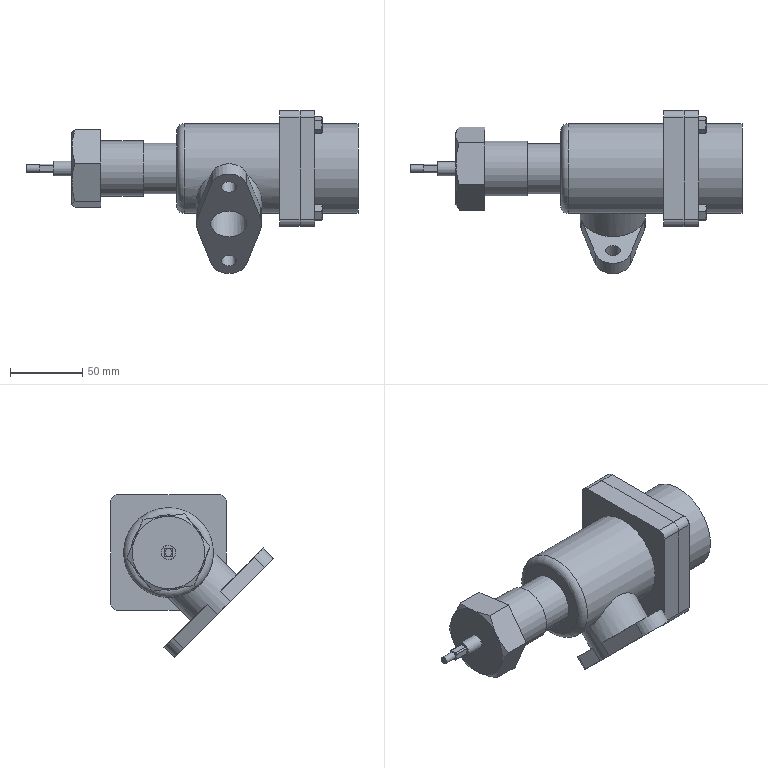Assembly | NX | mm | 19 component files | 19 solids | 279 faces | box 229 x 112.48 x 112.48 mm | volume 406841 mm3 | plane 116 | cylinder 79 | cone 79 | torus 3 | spline 1 | sphere 1 | commonest cylinder face diameters 6 x16 10 x13 16 x5 24 x4 2 x4 50 x3 40 x3 38 x3
Bill of materials:
GB-T6170_F-2000,M6x1 | 4 |  | Hexagonal prism with a central round through-bore; outer corners chamfered on both end faces; consistent with a hex nut form.
unnamed part 1 | 1 |  | Cylindrical plug or cap: a plain cylindrical body ending in a thin, tapered radial flange, followed by a short, smaller stepped disc that closes the end.
unnamed part 2 | 1 |  | Square flange with rounded corners and four corner holes. A larger hollow cylindrical boss sticks out from one face and two stepped, smaller cylindrical bosses stick out from the other face. A central round bore runs through.
unnamed part 3 | 1 |  | Flanged bushing: a thin annular flange with a smaller-diameter hollow cylindrical shank and a central through-bore.
unnamed part 4 | 1 |  | Flat circular ring with a rectangular cross-section, like a thin washer or spacer ring.
GB-T119.1-2000,6x24 | 4 |  | Parallel Pin, GB-T 119.1-2000,6x24
unnamed part 5 | 1 |  | Short thick-walled tubular sleeve with chamfered outer edges at both ends.
unnamed part 6 | 1 |  | Very thin flat annular ring, like a shim or thin washer.
unnamed part 7 | 1 |  | Housing body: a cylindrical main body with a square four-hole flange at one end, a stepped cylindrical spigot at the other end, and a side branch ending in an oval two-hole flange with a central bore, set at an angle.
unnamed part 8 | 1 |  | Slender stepped pin with a domed, hemispherical head at one end, a larger cylindrical collar near the head, and two reduced-diameter steps at the opposite tip.
unnamed part 9 | 1 |  | Hexagonal block with a large blind or stepped bore on one face and a smaller central through-hole visible from the opposite face. One end has chamfered corners.
unnamed part 10 | 1 |  | Thick flat annular ring or spacer with a rectangular cross-section.
unnamed part 11 | 1 |  | Hexagonal flange with a coaxial hollow cylindrical spigot. A short, narrower neck or undercut lies between the hex and the spigot, and a round through-bore runs through.
Mates:
1. touch align | valve_seat 1 face | valve_body 1 face
2. touch align | packing_gland 1 face | valve_body 1 face
3. touch align | gasket 1 face | valve_body 1 face
4. touch align | gasket 1 face | valve_body 1 face
5. touch align | packing 1 face | packing_gland 1 face
6. touch align | washer 1 face | packing_gland 1 face
7. touch align | nut 1 face | packing_gland 1 face
8. touch align | nut 1 face | packing_gland 1 face
9. touch align | valve 1 face | valve_stem 1 face
10. touch align | seal_ring 1 face | valve_stem 1 face
11. touch align | seal_ring 1 face | valve 1 face
12. touch align | lock_sleeve 1 face | valve_stem 1 face
13. touch align | GB-T6170_F-2000_M6x1 4 face | valve_seat 1 face
14. touch align | GB-T6170_F-2000_M6x1 4 face | valve_seat 1 face
15. touch align | GB-T119_1-2000_6x24 4 face | GB-T6170_F-2000_M6x1 4 face